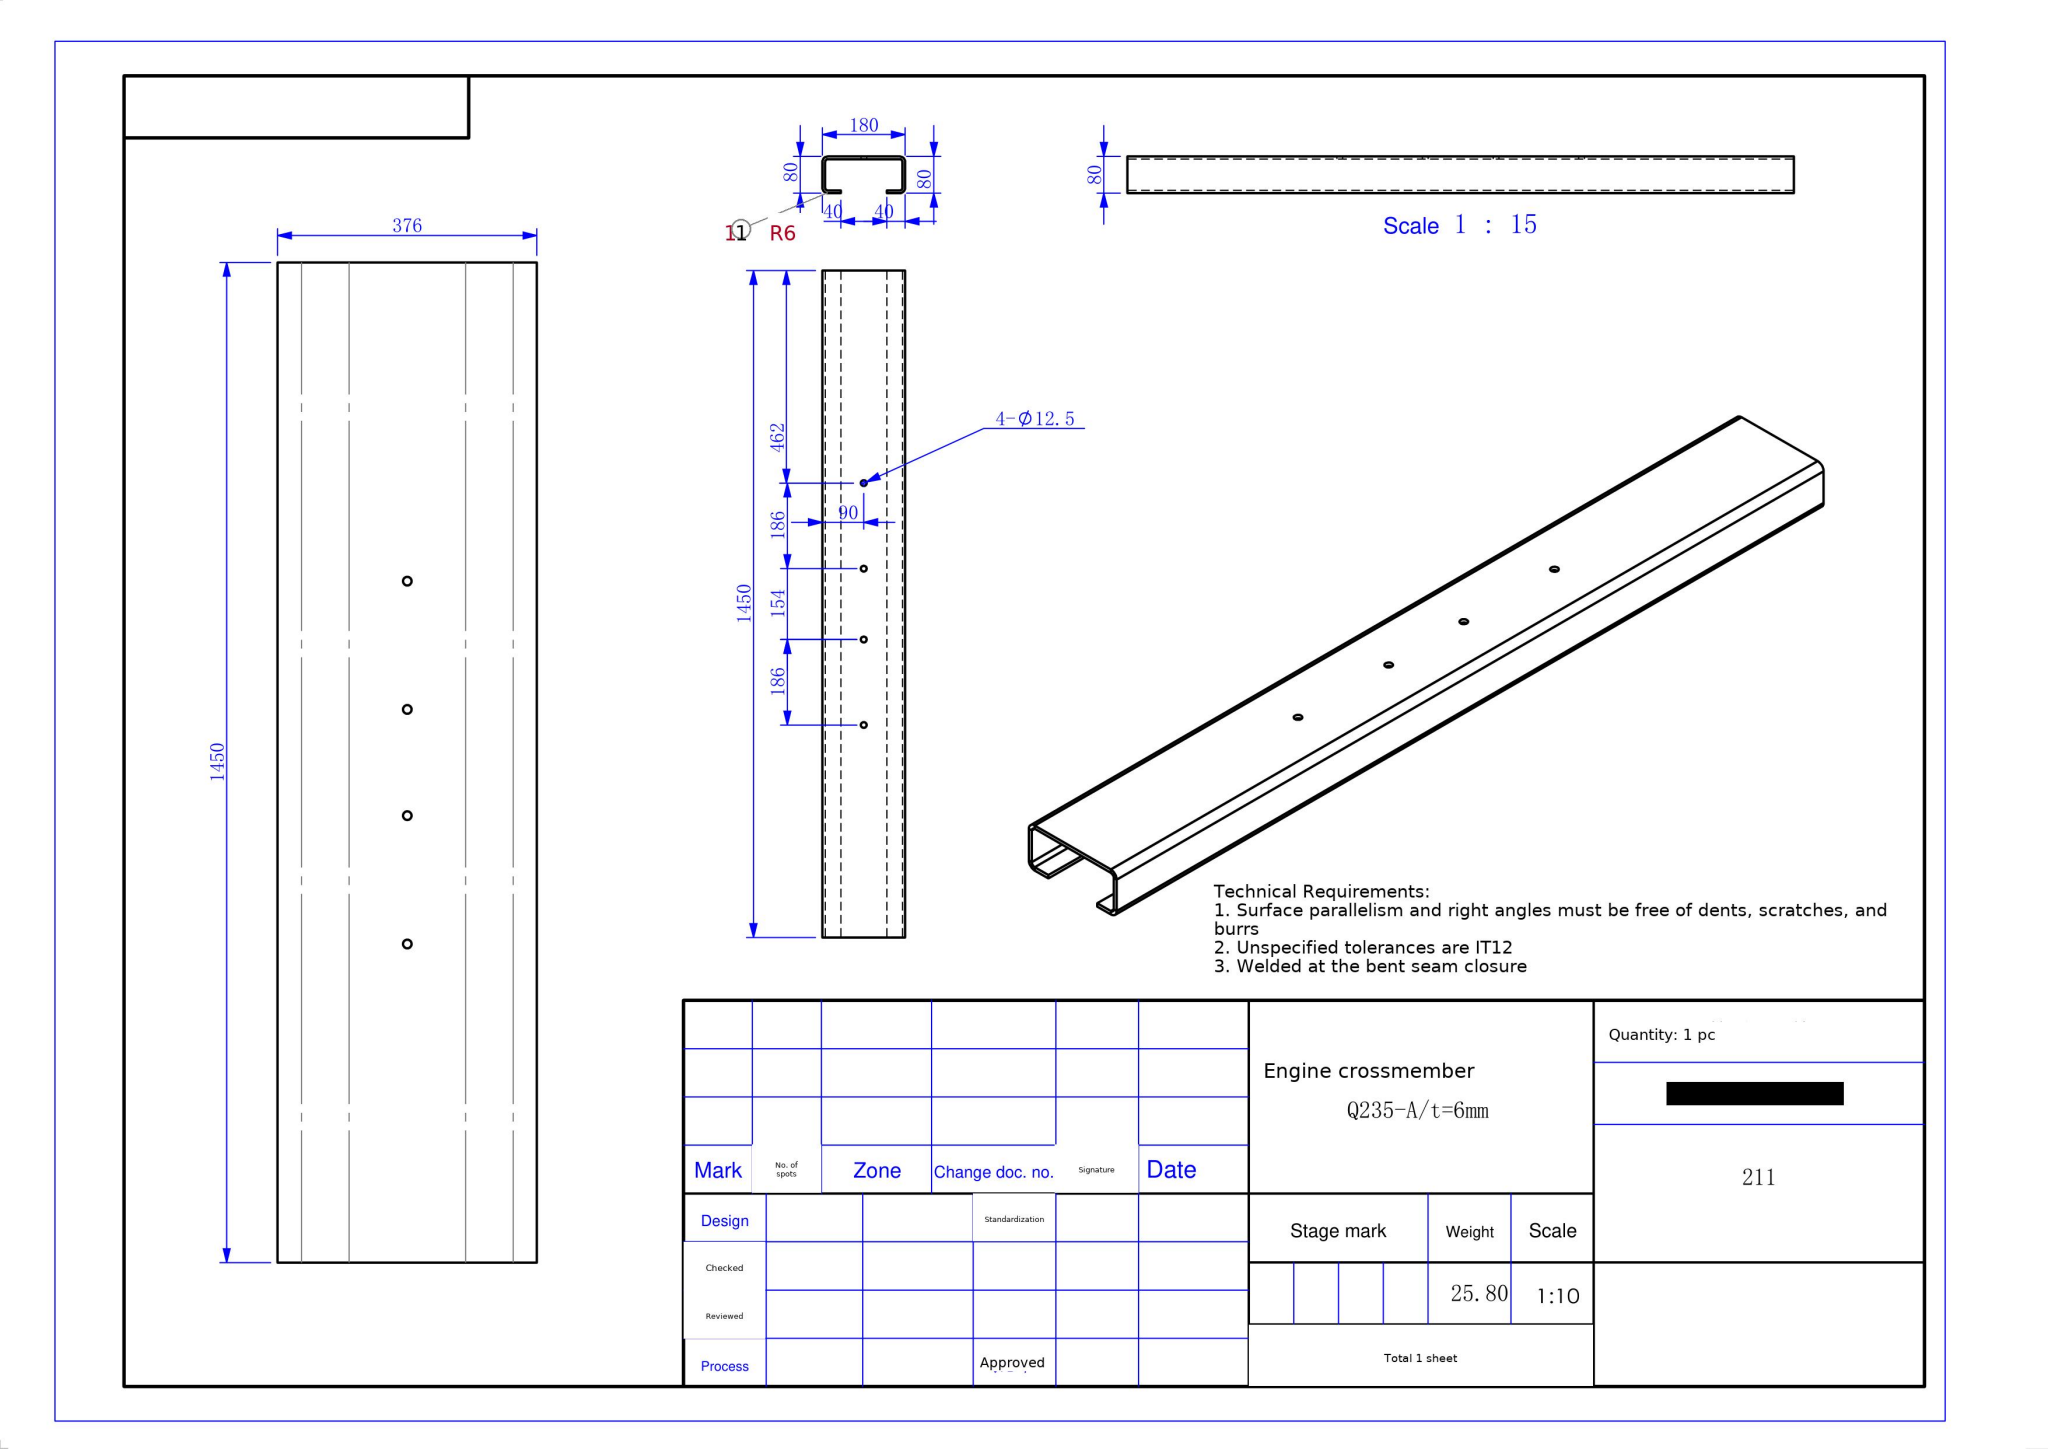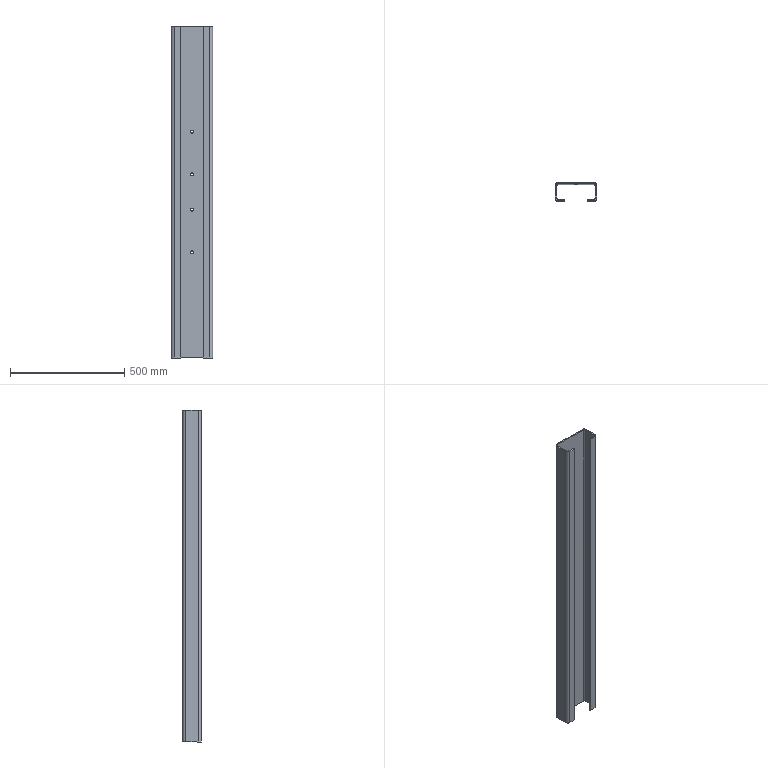Part | SolidWorks | mm | material Q235-A | 1 solid | 46 faces | box 180 x 80 x 1450 mm | volume 3307828 mm3 | plane 30 | cylinder 16 | commonest cylinder face diameters 12.5 x8 24 x4 12 x4